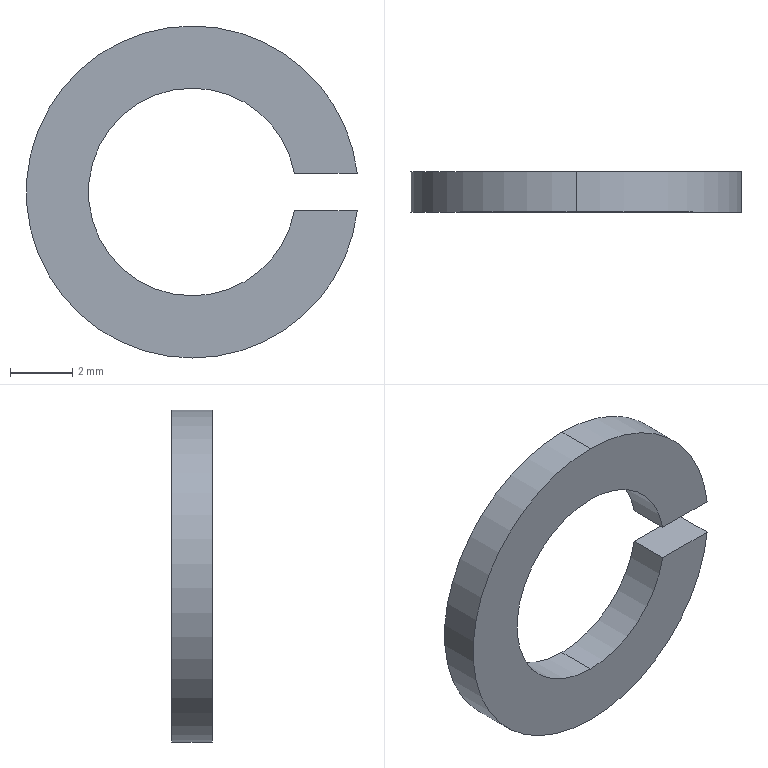Component | NX | WAVE_SPRING_WASHER_6_4 | 1 solid | 10 faces | box 10.65 x 1.3 x 10.68 mm | volume 68 mm3 | cylinder 6 | plane 4 | commonest cylinder face diameters 10.68 x3 6.68 x3
STEP:
#1=CARTESIAN_POINT('',(0.,0.,0.));
#2=DIRECTION('',(0.,0.,1.));
#3=DIRECTION('',(1.,0.,0.));
#4=AXIS2_PLACEMENT_3D('',#1,#2,#3);
#5=CARTESIAN_POINT('',(253.531,-87.,123.903));
#6=VERTEX_POINT('',#5);
#7=CARTESIAN_POINT('',(248.225,-87.,128.643));
#8=VERTEX_POINT('',#7);
#9=CARTESIAN_POINT('',(248.225,-87.,123.303));
#10=DIRECTION('',(0.,-1.,0.));
#11=DIRECTION('',(0.,0.,-1.));
#12=AXIS2_PLACEMENT_3D('',#9,#10,#11);
#13=CIRCLE('',#12,5.34);
#14=CARTESIAN_POINT('',(248.225,-87.65,123.303));
#15=DIRECTION('',(0.,-1.,0.));
#16=DIRECTION('',(0.,0.,1.));
#17=AXIS2_PLACEMENT_3D('',#14,#15,#16);
#18=CYLINDRICAL_SURFACE('',#17,5.34);
#19=CARTESIAN_POINT('',(3.142,-0.65));
#20=DIRECTION('',(1.,0.));
#21=VECTOR('',#20,1.);
#22=LINE('',#19,#21);
#23=(GEOMETRIC_REPRESENTATION_CONTEXT(2)PARAMETRIC_REPRESENTATION_CONTEXT()REPRESENTATION_CONTEXT('',''));
#24=DEFINITIONAL_REPRESENTATION('',(#22),#23);
#25=PCURVE('',#18,#24);
#26=CARTESIAN_POINT('',(251.565,-87.,123.303));
#27=DIRECTION('',(0.,1.,0.));
#28=DIRECTION('',(0.,0.,-1.));
#29=AXIS2_PLACEMENT_3D('',#26,#27,#28);
#30=PLANE('',#29);
#31=CARTESIAN_POINT('',(5.34,3.34));
#32=CARTESIAN_POINT('',(5.34,-5.909));
#33=CARTESIAN_POINT('',(-2.67,-1.285));
#34=CARTESIAN_POINT('',(-10.68,3.34));
#35=CARTESIAN_POINT('',(-2.67,7.965));
#36=CARTESIAN_POINT('',(5.34,12.589));
#37=CARTESIAN_POINT('',(5.34,3.34));
#38=(BOUNDED_CURVE()B_SPLINE_CURVE(2,(#31,#32,#33,#34,#35,#36,#37),.UNSPECIFIED.,.T.,.F.)B_SPLINE_CURVE_WITH_KNOTS((1,2,2,2,2,1),(-2.094,0.,2.094,4.189,6.283,8.378),.UNSPECIFIED.)CURVE()GEOMETRIC_REPRESENTATION_ITEM()RATIONAL_B_SPLINE_CURVE((1.,0.5,1.,0.5,1.,0.5,1.))REPRESENTATION_ITEM(''));
#39=(GEOMETRIC_REPRESENTATION_CONTEXT(2)PARAMETRIC_REPRESENTATION_CONTEXT()REPRESENTATION_CONTEXT('',''));
#40=DEFINITIONAL_REPRESENTATION('',(#38),#39);
#41=PCURVE('',#30,#40);
#42=SURFACE_CURVE('',#13,(#25,#41),.PCURVE_S1.);
#43=EDGE_CURVE('',#6,#8,#42,.T.);
#44=ORIENTED_EDGE('',*,*,#43,.T.);
#45=CARTESIAN_POINT('',(248.225,-88.3,128.643));
#46=VERTEX_POINT('',#45);
#47=CARTESIAN_POINT('',(248.225,-87.65,128.643));
#48=DIRECTION('',(0.,-1.,0.));
#49=VECTOR('',#48,1.);
#50=LINE('',#47,#49);
#51=CARTESIAN_POINT('',(6.283,0.));
#52=DIRECTION('',(0.,1.));
#53=VECTOR('',#52,1.);
#54=LINE('',#51,#53);
#55=(GEOMETRIC_REPRESENTATION_CONTEXT(2)PARAMETRIC_REPRESENTATION_CONTEXT()REPRESENTATION_CONTEXT('',''));
#56=DEFINITIONAL_REPRESENTATION('',(#54),#55);
#57=PCURVE('',#18,#56);
#58=CARTESIAN_POINT('',(248.225,-87.65,123.303));
#59=DIRECTION('',(0.,-1.,0.));
#60=DIRECTION('',(0.,0.,1.));
#61=AXIS2_PLACEMENT_3D('',#58,#59,#60);
#62=CYLINDRICAL_SURFACE('',#61,5.34);
#63=CARTESIAN_POINT('',(0.,0.));
#64=DIRECTION('',(0.,1.));
#65=VECTOR('',#64,1.);
#66=LINE('',#63,#65);
#67=(GEOMETRIC_REPRESENTATION_CONTEXT(2)PARAMETRIC_REPRESENTATION_CONTEXT()REPRESENTATION_CONTEXT('',''));
#68=DEFINITIONAL_REPRESENTATION('',(#66),#67);
#69=PCURVE('',#62,#68);
#70=SURFACE_CURVE('',#50,(#57,#69),.PCURVE_S1.);
#71=EDGE_CURVE('',#8,#46,#70,.T.);
#72=ORIENTED_EDGE('',*,*,#71,.T.);
#73=CARTESIAN_POINT('',(253.531,-88.3,123.903));
#74=VERTEX_POINT('',#73);
#75=CARTESIAN_POINT('',(248.225,-88.3,123.303));
#76=DIRECTION('',(0.,-1.,0.));
#77=DIRECTION('',(0.,0.,-1.));
#78=AXIS2_PLACEMENT_3D('',#75,#76,#77);
#79=CIRCLE('',#78,5.34);
#80=CARTESIAN_POINT('',(3.142,0.65));
#81=DIRECTION('',(1.,0.));
#82=VECTOR('',#81,1.);
#83=LINE('',#80,#82);
#84=(GEOMETRIC_REPRESENTATION_CONTEXT(2)PARAMETRIC_REPRESENTATION_CONTEXT()REPRESENTATION_CONTEXT('',''));
#85=DEFINITIONAL_REPRESENTATION('',(#83),#84);
#86=PCURVE('',#18,#85);
#87=CARTESIAN_POINT('',(251.565,-88.3,123.303));
#88=DIRECTION('',(0.,-1.,0.));
#89=DIRECTION('',(0.,0.,1.));
#90=AXIS2_PLACEMENT_3D('',#87,#88,#89);
#91=PLANE('',#90);
#92=CARTESIAN_POINT('',(0.,3.34));
#93=DIRECTION('',(-1.,0.));
#94=AXIS2_PLACEMENT_2D('',#92,#93);
#95=CIRCLE('',#94,5.34);
#96=(GEOMETRIC_REPRESENTATION_CONTEXT(2)PARAMETRIC_REPRESENTATION_CONTEXT()REPRESENTATION_CONTEXT('',''));
#97=DEFINITIONAL_REPRESENTATION('',(#95),#96);
#98=PCURVE('',#91,#97);
#99=SURFACE_CURVE('',#79,(#86,#98),.PCURVE_S1.);
#100=EDGE_CURVE('',#74,#46,#99,.T.);
#101=ORIENTED_EDGE('',*,*,#100,.F.);
#102=CARTESIAN_POINT('',(253.531,-87.65,123.903));
#103=DIRECTION('',(0.,-1.,0.));
#104=VECTOR('',#103,1.);
#105=LINE('',#102,#104);
#106=CARTESIAN_POINT('',(4.825,0.));
#107=DIRECTION('',(0.,1.));
#108=VECTOR('',#107,1.);
#109=LINE('',#106,#108);
#110=(GEOMETRIC_REPRESENTATION_CONTEXT(2)PARAMETRIC_REPRESENTATION_CONTEXT()REPRESENTATION_CONTEXT('',''));
#111=DEFINITIONAL_REPRESENTATION('',(#109),#110);
#112=PCURVE('',#18,#111);
#113=CARTESIAN_POINT('',(251.511,-88.3,123.903));
#114=DIRECTION('',(0.,0.,1.));
#115=DIRECTION('',(-1.,0.,0.));
#116=AXIS2_PLACEMENT_3D('',#113,#114,#115);
#117=PLANE('',#116);
#118=CARTESIAN_POINT('',(-2.021,-0.65));
#119=DIRECTION('',(0.,1.));
#120=VECTOR('',#119,1.);
#121=LINE('',#118,#120);
#122=(GEOMETRIC_REPRESENTATION_CONTEXT(2)PARAMETRIC_REPRESENTATION_CONTEXT()REPRESENTATION_CONTEXT('',''));
#123=DEFINITIONAL_REPRESENTATION('',(#121),#122);
#124=PCURVE('',#117,#123);
#125=SURFACE_CURVE('',#105,(#112,#124),.PCURVE_S1.);
#126=EDGE_CURVE('',#6,#74,#125,.T.);
#127=ORIENTED_EDGE('',*,*,#126,.F.);
#128=EDGE_LOOP('',(#44,#72,#101,#127));
#129=FACE_BOUND('',#128,.T.);
#130=ADVANCED_FACE('',(#129),#18,.T.);
#131=ORIENTED_EDGE('',*,*,#71,.F.);
#132=CARTESIAN_POINT('',(248.225,-87.,117.963));
#133=VERTEX_POINT('',#132);
#134=CARTESIAN_POINT('',(248.225,-87.,123.303));
#135=DIRECTION('',(0.,-1.,0.));
#136=DIRECTION('',(0.,0.,-1.));
#137=AXIS2_PLACEMENT_3D('',#134,#135,#136);
#138=CIRCLE('',#137,5.34);
#139=CARTESIAN_POINT('',(-3.142,-0.65));
#140=DIRECTION('',(1.,0.));
#141=VECTOR('',#140,1.);
#142=LINE('',#139,#141);
#143=(GEOMETRIC_REPRESENTATION_CONTEXT(2)PARAMETRIC_REPRESENTATION_CONTEXT()REPRESENTATION_CONTEXT('',''));
#144=DEFINITIONAL_REPRESENTATION('',(#142),#143);
#145=PCURVE('',#62,#144);
#146=CARTESIAN_POINT('',(5.34,3.34));
#147=CARTESIAN_POINT('',(5.34,-5.909));
#148=CARTESIAN_POINT('',(-2.67,-1.285));
#149=CARTESIAN_POINT('',(-10.68,3.34));
#150=CARTESIAN_POINT('',(-2.67,7.965));
#151=CARTESIAN_POINT('',(5.34,12.589));
#152=CARTESIAN_POINT('',(5.34,3.34));
#153=(BOUNDED_CURVE()B_SPLINE_CURVE(2,(#146,#147,#148,#149,#150,#151,#152),.UNSPECIFIED.,.T.,.F.)B_SPLINE_CURVE_WITH_KNOTS((1,2,2,2,2,1),(-2.094,0.,2.094,4.189,6.283,8.378),.UNSPECIFIED.)CURVE()GEOMETRIC_REPRESENTATION_ITEM()RATIONAL_B_SPLINE_CURVE((1.,0.5,1.,0.5,1.,0.5,1.))REPRESENTATION_ITEM(''));
#154=(GEOMETRIC_REPRESENTATION_CONTEXT(2)PARAMETRIC_REPRESENTATION_CONTEXT()REPRESENTATION_CONTEXT('',''));
#155=DEFINITIONAL_REPRESENTATION('',(#153),#154);
#156=PCURVE('',#30,#155);
#157=SURFACE_CURVE('',#138,(#145,#156),.PCURVE_S1.);
#158=EDGE_CURVE('',#8,#133,#157,.T.);
#159=ORIENTED_EDGE('',*,*,#158,.T.);
#160=CARTESIAN_POINT('',(248.225,-88.3,117.963));
#161=VERTEX_POINT('',#160);
#162=CARTESIAN_POINT('',(248.225,-87.65,117.963));
#163=DIRECTION('',(0.,-1.,0.));
#164=VECTOR('',#163,1.);
#165=LINE('',#162,#164);
#166=CARTESIAN_POINT('',(3.142,0.));
#167=DIRECTION('',(0.,1.));
#168=VECTOR('',#167,1.);
#169=LINE('',#166,#168);
#170=(GEOMETRIC_REPRESENTATION_CONTEXT(2)PARAMETRIC_REPRESENTATION_CONTEXT()REPRESENTATION_CONTEXT('',''));
#171=DEFINITIONAL_REPRESENTATION('',(#169),#170);
#172=PCURVE('',#62,#171);
#173=CARTESIAN_POINT('',(248.225,-87.65,123.303));
#174=DIRECTION('',(0.,-1.,0.));
#175=DIRECTION('',(0.,0.,1.));
#176=AXIS2_PLACEMENT_3D('',#173,#174,#175);
#177=CYLINDRICAL_SURFACE('',#176,5.34);
#178=CARTESIAN_POINT('',(3.142,0.));
#179=DIRECTION('',(0.,1.));
#180=VECTOR('',#179,1.);
#181=LINE('',#178,#180);
#182=(GEOMETRIC_REPRESENTATION_CONTEXT(2)PARAMETRIC_REPRESENTATION_CONTEXT()REPRESENTATION_CONTEXT('',''));
#183=DEFINITIONAL_REPRESENTATION('',(#181),#182);
#184=PCURVE('',#177,#183);
#185=SURFACE_CURVE('',#165,(#172,#184),.PCURVE_S1.);
#186=EDGE_CURVE('',#133,#161,#185,.T.);
#187=ORIENTED_EDGE('',*,*,#186,.T.);
#188=CARTESIAN_POINT('',(248.225,-88.3,123.303));
#189=DIRECTION('',(0.,-1.,0.));
#190=DIRECTION('',(0.,0.,-1.));
#191=AXIS2_PLACEMENT_3D('',#188,#189,#190);
#192=CIRCLE('',#191,5.34);
#193=CARTESIAN_POINT('',(-3.142,0.65));
#194=DIRECTION('',(1.,0.));
#195=VECTOR('',#194,1.);
#196=LINE('',#193,#195);
#197=(GEOMETRIC_REPRESENTATION_CONTEXT(2)PARAMETRIC_REPRESENTATION_CONTEXT()REPRESENTATION_CONTEXT('',''));
#198=DEFINITIONAL_REPRESENTATION('',(#196),#197);
#199=PCURVE('',#62,#198);
#200=CARTESIAN_POINT('',(0.,3.34));
#201=DIRECTION('',(-1.,0.));
#202=AXIS2_PLACEMENT_2D('',#200,#201);
#203=CIRCLE('',#202,5.34);
#204=(GEOMETRIC_REPRESENTATION_CONTEXT(2)PARAMETRIC_REPRESENTATION_CONTEXT()REPRESENTATION_CONTEXT('',''));
#205=DEFINITIONAL_REPRESENTATION('',(#203),#204);
#206=PCURVE('',#91,#205);
#207=SURFACE_CURVE('',#192,(#199,#206),.PCURVE_S1.);
#208=EDGE_CURVE('',#46,#161,#207,.T.);
#209=ORIENTED_EDGE('',*,*,#208,.F.);
#210=EDGE_LOOP('',(#131,#159,#187,#209));
#211=FACE_BOUND('',#210,.T.);
#212=ADVANCED_FACE('',(#211),#62,.T.);
#213=CARTESIAN_POINT('',(248.225,-87.,119.963));
#214=VERTEX_POINT('',#213);
#215=CARTESIAN_POINT('',(248.225,-88.3,119.963));
#216=VERTEX_POINT('',#215);
#217=CARTESIAN_POINT('',(248.225,-87.65,119.963));
#218=DIRECTION('',(0.,-1.,0.));
#219=VECTOR('',#218,1.);
#220=LINE('',#217,#219);
#221=CARTESIAN_POINT('',(248.225,-87.65,123.303));
#222=DIRECTION('',(0.,-1.,0.));
#223=DIRECTION('',(0.,0.,1.));
#224=AXIS2_PLACEMENT_3D('',#221,#222,#223);
#225=CYLINDRICAL_SURFACE('',#224,3.34);
#226=CARTESIAN_POINT('',(3.142,0.));
#227=DIRECTION('',(0.,1.));
#228=VECTOR('',#227,1.);
#229=LINE('',#226,#228);
#230=(GEOMETRIC_REPRESENTATION_CONTEXT(2)PARAMETRIC_REPRESENTATION_CONTEXT()REPRESENTATION_CONTEXT('',''));
#231=DEFINITIONAL_REPRESENTATION('',(#229),#230);
#232=PCURVE('',#225,#231);
#233=CARTESIAN_POINT('',(248.225,-87.65,123.303));
#234=DIRECTION('',(0.,-1.,0.));
#235=DIRECTION('',(0.,0.,1.));
#236=AXIS2_PLACEMENT_3D('',#233,#234,#235);
#237=CYLINDRICAL_SURFACE('',#236,3.34);
#238=CARTESIAN_POINT('',(3.142,0.));
#239=DIRECTION('',(0.,1.));
#240=VECTOR('',#239,1.);
#241=LINE('',#238,#240);
#242=(GEOMETRIC_REPRESENTATION_CONTEXT(2)PARAMETRIC_REPRESENTATION_CONTEXT()REPRESENTATION_CONTEXT('',''));
#243=DEFINITIONAL_REPRESENTATION('',(#241),#242);
#244=PCURVE('',#237,#243);
#245=SURFACE_CURVE('',#220,(#232,#244),.PCURVE_S1.);
#246=EDGE_CURVE('',#214,#216,#245,.T.);
#247=ORIENTED_EDGE('',*,*,#246,.T.);
#248=CARTESIAN_POINT('',(248.225,-88.3,126.643));
#249=VERTEX_POINT('',#248);
#250=CARTESIAN_POINT('',(248.225,-88.3,123.303));
#251=DIRECTION('',(0.,-1.,0.));
#252=DIRECTION('',(0.,0.,-1.));
#253=AXIS2_PLACEMENT_3D('',#250,#251,#252);
#254=CIRCLE('',#253,3.34);
#255=CARTESIAN_POINT('',(-3.142,0.65));
#256=DIRECTION('',(1.,0.));
#257=VECTOR('',#256,1.);
#258=LINE('',#255,#257);
#259=(GEOMETRIC_REPRESENTATION_CONTEXT(2)PARAMETRIC_REPRESENTATION_CONTEXT()REPRESENTATION_CONTEXT('',''));
#260=DEFINITIONAL_REPRESENTATION('',(#258),#259);
#261=PCURVE('',#225,#260);
#262=CARTESIAN_POINT('',(0.,3.34));
#263=DIRECTION('',(-1.,0.));
#264=AXIS2_PLACEMENT_2D('',#262,#263);
#265=CIRCLE('',#264,3.34);
#266=(GEOMETRIC_REPRESENTATION_CONTEXT(2)PARAMETRIC_REPRESENTATION_CONTEXT()REPRESENTATION_CONTEXT('',''));
#267=DEFINITIONAL_REPRESENTATION('',(#265),#266);
#268=PCURVE('',#91,#267);
#269=SURFACE_CURVE('',#254,(#261,#268),.PCURVE_S1.);
#270=EDGE_CURVE('',#249,#216,#269,.T.);
#271=ORIENTED_EDGE('',*,*,#270,.F.);
#272=CARTESIAN_POINT('',(248.225,-87.,126.643));
#273=VERTEX_POINT('',#272);
#274=CARTESIAN_POINT('',(248.225,-87.65,126.643));
#275=DIRECTION('',(0.,-1.,0.));
#276=VECTOR('',#275,1.);
#277=LINE('',#274,#276);
#278=CARTESIAN_POINT('',(0.,0.));
#279=DIRECTION('',(0.,1.));
#280=VECTOR('',#279,1.);
#281=LINE('',#278,#280);
#282=(GEOMETRIC_REPRESENTATION_CONTEXT(2)PARAMETRIC_REPRESENTATION_CONTEXT()REPRESENTATION_CONTEXT('',''));
#283=DEFINITIONAL_REPRESENTATION('',(#281),#282);
#284=PCURVE('',#225,#283);
#285=CARTESIAN_POINT('',(248.225,-87.65,123.303));
#286=DIRECTION('',(0.,-1.,0.));
#287=DIRECTION('',(0.,0.,1.));
#288=AXIS2_PLACEMENT_3D('',#285,#286,#287);
#289=CYLINDRICAL_SURFACE('',#288,3.34);
#290=CARTESIAN_POINT('',(6.283,0.));
#291=DIRECTION('',(0.,1.));
#292=VECTOR('',#291,1.);
#293=LINE('',#290,#292);
#294=(GEOMETRIC_REPRESENTATION_CONTEXT(2)PARAMETRIC_REPRESENTATION_CONTEXT()REPRESENTATION_CONTEXT('',''));
#295=DEFINITIONAL_REPRESENTATION('',(#293),#294);
#296=PCURVE('',#289,#295);
#297=SURFACE_CURVE('',#277,(#284,#296),.PCURVE_S1.);
#298=EDGE_CURVE('',#273,#249,#297,.T.);
#299=ORIENTED_EDGE('',*,*,#298,.F.);
#300=CARTESIAN_POINT('',(248.225,-87.,123.303));
#301=DIRECTION('',(0.,-1.,0.));
#302=DIRECTION('',(0.,0.,-1.));
#303=AXIS2_PLACEMENT_3D('',#300,#301,#302);
#304=CIRCLE('',#303,3.34);
#305=CARTESIAN_POINT('',(-3.142,-0.65));
#306=DIRECTION('',(1.,0.));
#307=VECTOR('',#306,1.);
#308=LINE('',#305,#307);
#309=(GEOMETRIC_REPRESENTATION_CONTEXT(2)PARAMETRIC_REPRESENTATION_CONTEXT()REPRESENTATION_CONTEXT('',''));
#310=DEFINITIONAL_REPRESENTATION('',(#308),#309);
#311=PCURVE('',#225,#310);
#312=CARTESIAN_POINT('',(3.34,3.34));
#313=CARTESIAN_POINT('',(3.34,-2.445));
#314=CARTESIAN_POINT('',(-1.67,0.4475));
#315=CARTESIAN_POINT('',(-6.68,3.34));
#316=CARTESIAN_POINT('',(-1.67,6.233));
#317=CARTESIAN_POINT('',(3.34,9.125));
#318=CARTESIAN_POINT('',(3.34,3.34));
#319=(BOUNDED_CURVE()B_SPLINE_CURVE(2,(#312,#313,#314,#315,#316,#317,#318),.UNSPECIFIED.,.T.,.F.)B_SPLINE_CURVE_WITH_KNOTS((1,2,2,2,2,1),(-2.094,0.,2.094,4.189,6.283,8.378),.UNSPECIFIED.)CURVE()GEOMETRIC_REPRESENTATION_ITEM()RATIONAL_B_SPLINE_CURVE((1.,0.5,1.,0.5,1.,0.5,1.))REPRESENTATION_ITEM(''));
#320=(GEOMETRIC_REPRESENTATION_CONTEXT(2)PARAMETRIC_REPRESENTATION_CONTEXT()REPRESENTATION_CONTEXT('',''));
#321=DEFINITIONAL_REPRESENTATION('',(#319),#320);
#322=PCURVE('',#30,#321);
#323=SURFACE_CURVE('',#304,(#311,#322),.PCURVE_S1.);
#324=EDGE_CURVE('',#273,#214,#323,.T.);
#325=ORIENTED_EDGE('',*,*,#324,.T.);
#326=EDGE_LOOP('',(#247,#271,#299,#325));
#327=FACE_BOUND('',#326,.F.);
#328=ADVANCED_FACE('',(#327),#225,.F.);
#329=CARTESIAN_POINT('',(251.511,-88.3,122.703));
#330=VERTEX_POINT('',#329);
#331=CARTESIAN_POINT('',(251.511,-87.,122.703));
#332=VERTEX_POINT('',#331);
#333=CARTESIAN_POINT('',(251.511,-88.3,122.703));
#334=DIRECTION('',(0.,1.,0.));
#335=VECTOR('',#334,1.);
#336=LINE('',#333,#335);
#337=CARTESIAN_POINT('',(4.532,0.65));
#338=DIRECTION('',(0.,-1.));
#339=VECTOR('',#338,1.);
#340=LINE('',#337,#339);
#341=(GEOMETRIC_REPRESENTATION_CONTEXT(2)PARAMETRIC_REPRESENTATION_CONTEXT()REPRESENTATION_CONTEXT('',''));
#342=DEFINITIONAL_REPRESENTATION('',(#340),#341);
#343=PCURVE('',#237,#342);
#344=CARTESIAN_POINT('',(251.511,-88.3,122.703));
#345=DIRECTION('',(0.,0.,-1.));
#346=DIRECTION('',(1.,0.,0.));
#347=AXIS2_PLACEMENT_3D('',#344,#345,#346);
#348=PLANE('',#347);
#349=CARTESIAN_POINT('',(0.,0.));
#350=DIRECTION('',(0.,-1.));
#351=VECTOR('',#350,1.);
#352=LINE('',#349,#351);
#353=(GEOMETRIC_REPRESENTATION_CONTEXT(2)PARAMETRIC_REPRESENTATION_CONTEXT()REPRESENTATION_CONTEXT('',''));
#354=DEFINITIONAL_REPRESENTATION('',(#352),#353);
#355=PCURVE('',#348,#354);
#356=SURFACE_CURVE('',#336,(#343,#355),.PCURVE_S1.);
#357=EDGE_CURVE('',#330,#332,#356,.T.);
#358=ORIENTED_EDGE('',*,*,#357,.F.);
#359=CARTESIAN_POINT('',(248.225,-88.3,123.303));
#360=DIRECTION('',(0.,-1.,0.));
#361=DIRECTION('',(0.,0.,-1.));
#362=AXIS2_PLACEMENT_3D('',#359,#360,#361);
#363=CIRCLE('',#362,3.34);
#364=CARTESIAN_POINT('',(3.142,0.65));
#365=DIRECTION('',(1.,0.));
#366=VECTOR('',#365,1.);
#367=LINE('',#364,#366);
#368=(GEOMETRIC_REPRESENTATION_CONTEXT(2)PARAMETRIC_REPRESENTATION_CONTEXT()REPRESENTATION_CONTEXT('',''));
#369=DEFINITIONAL_REPRESENTATION('',(#367),#368);
#370=PCURVE('',#237,#369);
#371=CARTESIAN_POINT('',(0.,3.34));
#372=DIRECTION('',(-1.,0.));
#373=AXIS2_PLACEMENT_2D('',#371,#372);
#374=CIRCLE('',#373,3.34);
#375=(GEOMETRIC_REPRESENTATION_CONTEXT(2)PARAMETRIC_REPRESENTATION_CONTEXT()REPRESENTATION_CONTEXT('',''));
#376=DEFINITIONAL_REPRESENTATION('',(#374),#375);
#377=PCURVE('',#91,#376);
#378=SURFACE_CURVE('',#363,(#370,#377),.PCURVE_S1.);
#379=EDGE_CURVE('',#216,#330,#378,.T.);
#380=ORIENTED_EDGE('',*,*,#379,.F.);
#381=ORIENTED_EDGE('',*,*,#246,.F.);
#382=CARTESIAN_POINT('',(248.225,-87.,123.303));
#383=DIRECTION('',(0.,-1.,0.));
#384=DIRECTION('',(0.,0.,-1.));
#385=AXIS2_PLACEMENT_3D('',#382,#383,#384);
#386=CIRCLE('',#385,3.34);
#387=CARTESIAN_POINT('',(3.142,-0.65));
#388=DIRECTION('',(1.,0.));
#389=VECTOR('',#388,1.);
#390=LINE('',#387,#389);
#391=(GEOMETRIC_REPRESENTATION_CONTEXT(2)PARAMETRIC_REPRESENTATION_CONTEXT()REPRESENTATION_CONTEXT('',''));
#392=DEFINITIONAL_REPRESENTATION('',(#390),#391);
#393=PCURVE('',#237,#392);
#394=CARTESIAN_POINT('',(3.34,3.34));
#395=CARTESIAN_POINT('',(3.34,-2.445));
#396=CARTESIAN_POINT('',(-1.67,0.4475));
#397=CARTESIAN_POINT('',(-6.68,3.34));
#398=CARTESIAN_POINT('',(-1.67,6.233));
#399=CARTESIAN_POINT('',(3.34,9.125));
#400=CARTESIAN_POINT('',(3.34,3.34));
#401=(BOUNDED_CURVE()B_SPLINE_CURVE(2,(#394,#395,#396,#397,#398,#399,#400),.UNSPECIFIED.,.T.,.F.)B_SPLINE_CURVE_WITH_KNOTS((1,2,2,2,2,1),(-2.094,0.,2.094,4.189,6.283,8.378),.UNSPECIFIED.)CURVE()GEOMETRIC_REPRESENTATION_ITEM()RATIONAL_B_SPLINE_CURVE((1.,0.5,1.,0.5,1.,0.5,1.))REPRESENTATION_ITEM(''));
#402=(GEOMETRIC_REPRESENTATION_CONTEXT(2)PARAMETRIC_REPRESENTATION_CONTEXT()REPRESENTATION_CONTEXT('',''));
#403=DEFINITIONAL_REPRESENTATION('',(#401),#402);
#404=PCURVE('',#30,#403);
#405=SURFACE_CURVE('',#386,(#393,#404),.PCURVE_S1.);
#406=EDGE_CURVE('',#214,#332,#405,.T.);
#407=ORIENTED_EDGE('',*,*,#406,.T.);
#408=EDGE_LOOP('',(#358,#380,#381,#407));
#409=FACE_BOUND('',#408,.F.);
#410=ADVANCED_FACE('',(#409),#237,.F.);
#411=CARTESIAN_POINT('',(251.511,-88.3,123.903));
#412=VERTEX_POINT('',#411);
#413=CARTESIAN_POINT('',(248.225,-88.3,123.303));
#414=DIRECTION('',(0.,-1.,0.));
#415=DIRECTION('',(0.,0.,-1.));
#416=AXIS2_PLACEMENT_3D('',#413,#414,#415);
#417=CIRCLE('',#416,3.34);
#418=CARTESIAN_POINT('',(3.142,0.65));
#419=DIRECTION('',(1.,0.));
#420=VECTOR('',#419,1.);
#421=LINE('',#418,#420);
#422=(GEOMETRIC_REPRESENTATION_CONTEXT(2)PARAMETRIC_REPRESENTATION_CONTEXT()REPRESENTATION_CONTEXT('',''));
#423=DEFINITIONAL_REPRESENTATION('',(#421),#422);
#424=PCURVE('',#289,#423);
#425=CARTESIAN_POINT('',(0.,3.34));
#426=DIRECTION('',(-1.,0.));
#427=AXIS2_PLACEMENT_2D('',#425,#426);
#428=CIRCLE('',#427,3.34);
#429=(GEOMETRIC_REPRESENTATION_CONTEXT(2)PARAMETRIC_REPRESENTATION_CONTEXT()REPRESENTATION_CONTEXT('',''));
#430=DEFINITIONAL_REPRESENTATION('',(#428),#429);
#431=PCURVE('',#91,#430);
#432=SURFACE_CURVE('',#417,(#424,#431),.PCURVE_S1.);
#433=EDGE_CURVE('',#412,#249,#432,.T.);
#434=ORIENTED_EDGE('',*,*,#433,.F.);
#435=CARTESIAN_POINT('',(251.511,-87.,123.903));
#436=VERTEX_POINT('',#435);
#437=CARTESIAN_POINT('',(251.511,-88.3,123.903));
#438=DIRECTION('',(0.,1.,0.));
#439=VECTOR('',#438,1.);
#440=LINE('',#437,#439);
#441=CARTESIAN_POINT('',(4.893,0.65));
#442=DIRECTION('',(0.,-1.));
#443=VECTOR('',#442,1.);
#444=LINE('',#441,#443);
#445=(GEOMETRIC_REPRESENTATION_CONTEXT(2)PARAMETRIC_REPRESENTATION_CONTEXT()REPRESENTATION_CONTEXT('',''));
#446=DEFINITIONAL_REPRESENTATION('',(#444),#445);
#447=PCURVE('',#289,#446);
#448=CARTESIAN_POINT('',(0.,0.));
#449=DIRECTION('',(0.,-1.));
#450=VECTOR('',#449,1.);
#451=LINE('',#448,#450);
#452=(GEOMETRIC_REPRESENTATION_CONTEXT(2)PARAMETRIC_REPRESENTATION_CONTEXT()REPRESENTATION_CONTEXT('',''));
#453=DEFINITIONAL_REPRESENTATION('',(#451),#452);
#454=PCURVE('',#117,#453);
#455=SURFACE_CURVE('',#440,(#447,#454),.PCURVE_S1.);
#456=EDGE_CURVE('',#412,#436,#455,.T.);
#457=ORIENTED_EDGE('',*,*,#456,.T.);
#458=CARTESIAN_POINT('',(248.225,-87.,123.303));
#459=DIRECTION('',(0.,-1.,0.));
#460=DIRECTION('',(0.,0.,-1.));
#461=AXIS2_PLACEMENT_3D('',#458,#459,#460);
#462=CIRCLE('',#461,3.34);
#463=CARTESIAN_POINT('',(3.142,-0.65));
#464=DIRECTION('',(1.,0.));
#465=VECTOR('',#464,1.);
#466=LINE('',#463,#465);
#467=(GEOMETRIC_REPRESENTATION_CONTEXT(2)PARAMETRIC_REPRESENTATION_CONTEXT()REPRESENTATION_CONTEXT('',''));
#468=DEFINITIONAL_REPRESENTATION('',(#466),#467);
#469=PCURVE('',#289,#468);
#470=CARTESIAN_POINT('',(3.34,3.34));
#471=CARTESIAN_POINT('',(3.34,-2.445));
#472=CARTESIAN_POINT('',(-1.67,0.4475));
#473=CARTESIAN_POINT('',(-6.68,3.34));
#474=CARTESIAN_POINT('',(-1.67,6.233));
#475=CARTESIAN_POINT('',(3.34,9.125));
#476=CARTESIAN_POINT('',(3.34,3.34));
#477=(BOUNDED_CURVE()B_SPLINE_CURVE(2,(#470,#471,#472,#473,#474,#475,#476),.UNSPECIFIED.,.T.,.F.)B_SPLINE_CURVE_WITH_KNOTS((1,2,2,2,2,1),(-2.094,0.,2.094,4.189,6.283,8.378),.UNSPECIFIED.)CURVE()GEOMETRIC_REPRESENTATION_ITEM()RATIONAL_B_SPLINE_CURVE((1.,0.5,1.,0.5,1.,0.5,1.))REPRESENTATION_ITEM(''));
#478=(GEOMETRIC_REPRESENTATION_CONTEXT(2)PARAMETRIC_REPRESENTATION_CONTEXT()REPRESENTATION_CONTEXT('',''));
#479=DEFINITIONAL_REPRESENTATION('',(#477),#478);
#480=PCURVE('',#30,#479);
#481=SURFACE_CURVE('',#462,(#469,#480),.PCURVE_S1.);
#482=EDGE_CURVE('',#436,#273,#481,.T.);
#483=ORIENTED_EDGE('',*,*,#482,.T.);
#484=ORIENTED_EDGE('',*,*,#298,.T.);
#485=EDGE_LOOP('',(#434,#457,#483,#484));
#486=FACE_BOUND('',#485,.F.);
#487=ADVANCED_FACE('',(#486),#289,.F.);
#488=CARTESIAN_POINT('',(253.531,-88.3,122.703));
#489=VERTEX_POINT('',#488);
#490=CARTESIAN_POINT('',(251.511,-88.3,122.703));
#491=DIRECTION('',(-1.,0.,0.));
#492=VECTOR('',#491,1.);
#493=LINE('',#490,#492);
#494=CARTESIAN_POINT('',(-0.6,0.05433));
#495=DIRECTION('',(0.,1.));
#496=VECTOR('',#495,1.);
#497=LINE('',#494,#496);
#498=(GEOMETRIC_REPRESENTATION_CONTEXT(2)PARAMETRIC_REPRESENTATION_CONTEXT()REPRESENTATION_CONTEXT('',''));
#499=DEFINITIONAL_REPRESENTATION('',(#497),#498);
#500=PCURVE('',#91,#499);
#501=CARTESIAN_POINT('',(0.,0.));
#502=DIRECTION('',(-1.,0.));
#503=VECTOR('',#502,1.);
#504=LINE('',#501,#503);
#505=(GEOMETRIC_REPRESENTATION_CONTEXT(2)PARAMETRIC_REPRESENTATION_CONTEXT()REPRESENTATION_CONTEXT('',''));
#506=DEFINITIONAL_REPRESENTATION('',(#504),#505);
#507=PCURVE('',#348,#506);
#508=SURFACE_CURVE('',#493,(#500,#507),.PCURVE_S1.);
#509=EDGE_CURVE('',#489,#330,#508,.T.);
#510=ORIENTED_EDGE('',*,*,#509,.T.);
#511=ORIENTED_EDGE('',*,*,#379,.F.);
#512=ORIENTED_EDGE('',*,*,#270,.F.);
#513=ORIENTED_EDGE('',*,*,#433,.F.);
#514=CARTESIAN_POINT('',(251.511,-88.3,123.903));
#515=DIRECTION('',(1.,0.,0.));
#516=VECTOR('',#515,1.);
#517=LINE('',#514,#516);
#518=CARTESIAN_POINT('',(0.6,0.05433));
#519=DIRECTION('',(0.,-1.));
#520=VECTOR('',#519,1.);
#521=LINE('',#518,#520);
#522=(GEOMETRIC_REPRESENTATION_CONTEXT(2)PARAMETRIC_REPRESENTATION_CONTEXT()REPRESENTATION_CONTEXT('',''));
#523=DEFINITIONAL_REPRESENTATION('',(#521),#522);
#524=PCURVE('',#91,#523);
#525=CARTESIAN_POINT('',(0.,0.));
#526=DIRECTION('',(-1.,0.));
#527=VECTOR('',#526,1.);
#528=LINE('',#525,#527);
#529=(GEOMETRIC_REPRESENTATION_CONTEXT(2)PARAMETRIC_REPRESENTATION_CONTEXT()REPRESENTATION_CONTEXT('',''));
#530=DEFINITIONAL_REPRESENTATION('',(#528),#529);
#531=PCURVE('',#117,#530);
#532=SURFACE_CURVE('',#517,(#524,#531),.PCURVE_S1.);
#533=EDGE_CURVE('',#412,#74,#532,.T.);
#534=ORIENTED_EDGE('',*,*,#533,.T.);
#535=ORIENTED_EDGE('',*,*,#100,.T.);
#536=ORIENTED_EDGE('',*,*,#208,.T.);
#537=CARTESIAN_POINT('',(248.225,-88.3,123.303));
#538=DIRECTION('',(0.,-1.,0.));
#539=DIRECTION('',(0.,0.,-1.));
#540=AXIS2_PLACEMENT_3D('',#537,#538,#539);
#541=CIRCLE('',#540,5.34);
#542=CARTESIAN_POINT('',(0.,3.34));
#543=DIRECTION('',(-1.,0.));
#544=AXIS2_PLACEMENT_2D('',#542,#543);
#545=CIRCLE('',#544,5.34);
#546=(GEOMETRIC_REPRESENTATION_CONTEXT(2)PARAMETRIC_REPRESENTATION_CONTEXT()REPRESENTATION_CONTEXT('',''));
#547=DEFINITIONAL_REPRESENTATION('',(#545),#546);
#548=PCURVE('',#91,#547);
#549=CARTESIAN_POINT('',(3.142,0.65));
#550=DIRECTION('',(1.,0.));
#551=VECTOR('',#550,1.);
#552=LINE('',#549,#551);
#553=(GEOMETRIC_REPRESENTATION_CONTEXT(2)PARAMETRIC_REPRESENTATION_CONTEXT()REPRESENTATION_CONTEXT('',''));
#554=DEFINITIONAL_REPRESENTATION('',(#552),#553);
#555=PCURVE('',#177,#554);
#556=SURFACE_CURVE('',#541,(#548,#555),.PCURVE_S1.);
#557=EDGE_CURVE('',#161,#489,#556,.T.);
#558=ORIENTED_EDGE('',*,*,#557,.T.);
#559=EDGE_LOOP('',(#510,#511,#512,#513,#534,#535,#536,#558));
#560=FACE_BOUND('',#559,.T.);
#561=ADVANCED_FACE('',(#560),#91,.T.);
#562=ORIENTED_EDGE('',*,*,#186,.F.);
#563=CARTESIAN_POINT('',(253.531,-87.,122.703));
#564=VERTEX_POINT('',#563);
#565=CARTESIAN_POINT('',(248.225,-87.,123.303));
#566=DIRECTION('',(0.,-1.,0.));
#567=DIRECTION('',(0.,0.,-1.));
#568=AXIS2_PLACEMENT_3D('',#565,#566,#567);
#569=CIRCLE('',#568,5.34);
#570=CARTESIAN_POINT('',(3.142,-0.65));
#571=DIRECTION('',(1.,0.));
#572=VECTOR('',#571,1.);
#573=LINE('',#570,#572);
#574=(GEOMETRIC_REPRESENTATION_CONTEXT(2)PARAMETRIC_REPRESENTATION_CONTEXT()REPRESENTATION_CONTEXT('',''));
#575=DEFINITIONAL_REPRESENTATION('',(#573),#574);
#576=PCURVE('',#177,#575);
#577=CARTESIAN_POINT('',(5.34,3.34));
#578=CARTESIAN_POINT('',(5.34,-5.909));
#579=CARTESIAN_POINT('',(-2.67,-1.285));
#580=CARTESIAN_POINT('',(-10.68,3.34));
#581=CARTESIAN_POINT('',(-2.67,7.965));
#582=CARTESIAN_POINT('',(5.34,12.589));
#583=CARTESIAN_POINT('',(5.34,3.34));
#584=(BOUNDED_CURVE()B_SPLINE_CURVE(2,(#577,#578,#579,#580,#581,#582,#583),.UNSPECIFIED.,.T.,.F.)B_SPLINE_CURVE_WITH_KNOTS((1,2,2,2,2,1),(-2.094,0.,2.094,4.189,6.283,8.378),.UNSPECIFIED.)CURVE()GEOMETRIC_REPRESENTATION_ITEM()RATIONAL_B_SPLINE_CURVE((1.,0.5,1.,0.5,1.,0.5,1.))REPRESENTATION_ITEM(''));
#585=(GEOMETRIC_REPRESENTATION_CONTEXT(2)PARAMETRIC_REPRESENTATION_CONTEXT()REPRESENTATION_CONTEXT('',''));
#586=DEFINITIONAL_REPRESENTATION('',(#584),#585);
#587=PCURVE('',#30,#586);
#588=SURFACE_CURVE('',#569,(#576,#587),.PCURVE_S1.);
#589=EDGE_CURVE('',#133,#564,#588,.T.);
#590=ORIENTED_EDGE('',*,*,#589,.T.);
#591=CARTESIAN_POINT('',(253.531,-87.65,122.703));
#592=DIRECTION('',(0.,1.,0.));
#593=VECTOR('',#592,1.);
#594=LINE('',#591,#593);
#595=CARTESIAN_POINT('',(4.6,0.));
#596=DIRECTION('',(0.,-1.));
#597=VECTOR('',#596,1.);
#598=LINE('',#595,#597);
#599=(GEOMETRIC_REPRESENTATION_CONTEXT(2)PARAMETRIC_REPRESENTATION_CONTEXT()REPRESENTATION_CONTEXT('',''));
#600=DEFINITIONAL_REPRESENTATION('',(#598),#599);
#601=PCURVE('',#177,#600);
#602=CARTESIAN_POINT('',(2.021,-0.65));
#603=DIRECTION('',(0.,-1.));
#604=VECTOR('',#603,1.);
#605=LINE('',#602,#604);
#606=(GEOMETRIC_REPRESENTATION_CONTEXT(2)PARAMETRIC_REPRESENTATION_CONTEXT()REPRESENTATION_CONTEXT('',''));
#607=DEFINITIONAL_REPRESENTATION('',(#605),#606);
#608=PCURVE('',#348,#607);
#609=SURFACE_CURVE('',#594,(#601,#608),.PCURVE_S1.);
#610=EDGE_CURVE('',#489,#564,#609,.T.);
#611=ORIENTED_EDGE('',*,*,#610,.F.);
#612=ORIENTED_EDGE('',*,*,#557,.F.);
#613=EDGE_LOOP('',(#562,#590,#611,#612));
#614=FACE_BOUND('',#613,.T.);
#615=ADVANCED_FACE('',(#614),#177,.T.);
#616=CARTESIAN_POINT('',(251.565,-87.,122.703));
#617=DIRECTION('',(-1.,0.,0.));
#618=VECTOR('',#617,1.);
#619=LINE('',#616,#618);
#620=CARTESIAN_POINT('',(0.6,0.));
#621=DIRECTION('',(0.,1.));
#622=VECTOR('',#621,1.);
#623=LINE('',#620,#622);
#624=(GEOMETRIC_REPRESENTATION_CONTEXT(2)PARAMETRIC_REPRESENTATION_CONTEXT()REPRESENTATION_CONTEXT('',''));
#625=DEFINITIONAL_REPRESENTATION('',(#623),#624);
#626=PCURVE('',#30,#625);
#627=CARTESIAN_POINT('',(0.05433,-1.3));
#628=DIRECTION('',(-1.,0.));
#629=VECTOR('',#628,1.);
#630=LINE('',#627,#629);
#631=(GEOMETRIC_REPRESENTATION_CONTEXT(2)PARAMETRIC_REPRESENTATION_CONTEXT()REPRESENTATION_CONTEXT('',''));
#632=DEFINITIONAL_REPRESENTATION('',(#630),#631);
#633=PCURVE('',#348,#632);
#634=SURFACE_CURVE('',#619,(#626,#633),.PCURVE_S1.);
#635=EDGE_CURVE('',#564,#332,#634,.T.);
#636=ORIENTED_EDGE('',*,*,#635,.F.);
#637=ORIENTED_EDGE('',*,*,#589,.F.);
#638=ORIENTED_EDGE('',*,*,#158,.F.);
#639=ORIENTED_EDGE('',*,*,#43,.F.);
#640=CARTESIAN_POINT('',(251.511,-87.,123.903));
#641=DIRECTION('',(1.,0.,0.));
#642=VECTOR('',#641,1.);
#643=LINE('',#640,#642);
#644=CARTESIAN_POINT('',(-0.6,0.05433));
#645=DIRECTION('',(0.,-1.));
#646=VECTOR('',#645,1.);
#647=LINE('',#644,#646);
#648=(GEOMETRIC_REPRESENTATION_CONTEXT(2)PARAMETRIC_REPRESENTATION_CONTEXT()REPRESENTATION_CONTEXT('',''));
#649=DEFINITIONAL_REPRESENTATION('',(#647),#648);
#650=PCURVE('',#30,#649);
#651=CARTESIAN_POINT('',(0.,-1.3));
#652=DIRECTION('',(-1.,0.));
#653=VECTOR('',#652,1.);
#654=LINE('',#651,#653);
#655=(GEOMETRIC_REPRESENTATION_CONTEXT(2)PARAMETRIC_REPRESENTATION_CONTEXT()REPRESENTATION_CONTEXT('',''));
#656=DEFINITIONAL_REPRESENTATION('',(#654),#655);
#657=PCURVE('',#117,#656);
#658=SURFACE_CURVE('',#643,(#650,#657),.PCURVE_S1.);
#659=EDGE_CURVE('',#436,#6,#658,.T.);
#660=ORIENTED_EDGE('',*,*,#659,.F.);
#661=ORIENTED_EDGE('',*,*,#482,.T.);
#662=ORIENTED_EDGE('',*,*,#324,.T.);
#663=ORIENTED_EDGE('',*,*,#406,.T.);
#664=EDGE_LOOP('',(#636,#637,#638,#639,#660,#661,#662,#663));
#665=FACE_BOUND('',#664,.T.);
#666=ADVANCED_FACE('',(#665),#30,.T.);
#667=ORIENTED_EDGE('',*,*,#126,.T.);
#668=ORIENTED_EDGE('',*,*,#533,.F.);
#669=ORIENTED_EDGE('',*,*,#456,.T.);
#670=ORIENTED_EDGE('',*,*,#659,.T.);
#671=EDGE_LOOP('',(#667,#668,#669,#670));
#672=FACE_BOUND('',#671,.T.);
#673=ADVANCED_FACE('',(#672),#117,.F.);
#674=ORIENTED_EDGE('',*,*,#610,.T.);
#675=ORIENTED_EDGE('',*,*,#635,.T.);
#676=ORIENTED_EDGE('',*,*,#357,.F.);
#677=ORIENTED_EDGE('',*,*,#509,.F.);
#678=EDGE_LOOP('',(#674,#675,#676,#677));
#679=FACE_BOUND('',#678,.T.);
#680=ADVANCED_FACE('',(#679),#348,.F.);
#681=CLOSED_SHELL('',(#130,#212,#328,#410,#487,#561,#615,#666,#673,#680));
#682=MANIFOLD_SOLID_BREP('',#681);
#683=(LENGTH_UNIT()NAMED_UNIT(*)SI_UNIT(.MILLI.,.METRE.));
#684=UNCERTAINTY_MEASURE_WITH_UNIT(LENGTH_MEASURE(0.0000001),#683,'','');
#685=(NAMED_UNIT(*)PLANE_ANGLE_UNIT()SI_UNIT($,.RADIAN.));
#686=(NAMED_UNIT(*)SI_UNIT($,.STERADIAN.)SOLID_ANGLE_UNIT());
#687=(GEOMETRIC_REPRESENTATION_CONTEXT(3)GLOBAL_UNCERTAINTY_ASSIGNED_CONTEXT((#684))GLOBAL_UNIT_ASSIGNED_CONTEXT((#683,#685,#686))REPRESENTATION_CONTEXT('',''));
#688=ADVANCED_BREP_SHAPE_REPRESENTATION('',(#4,#682),#687);